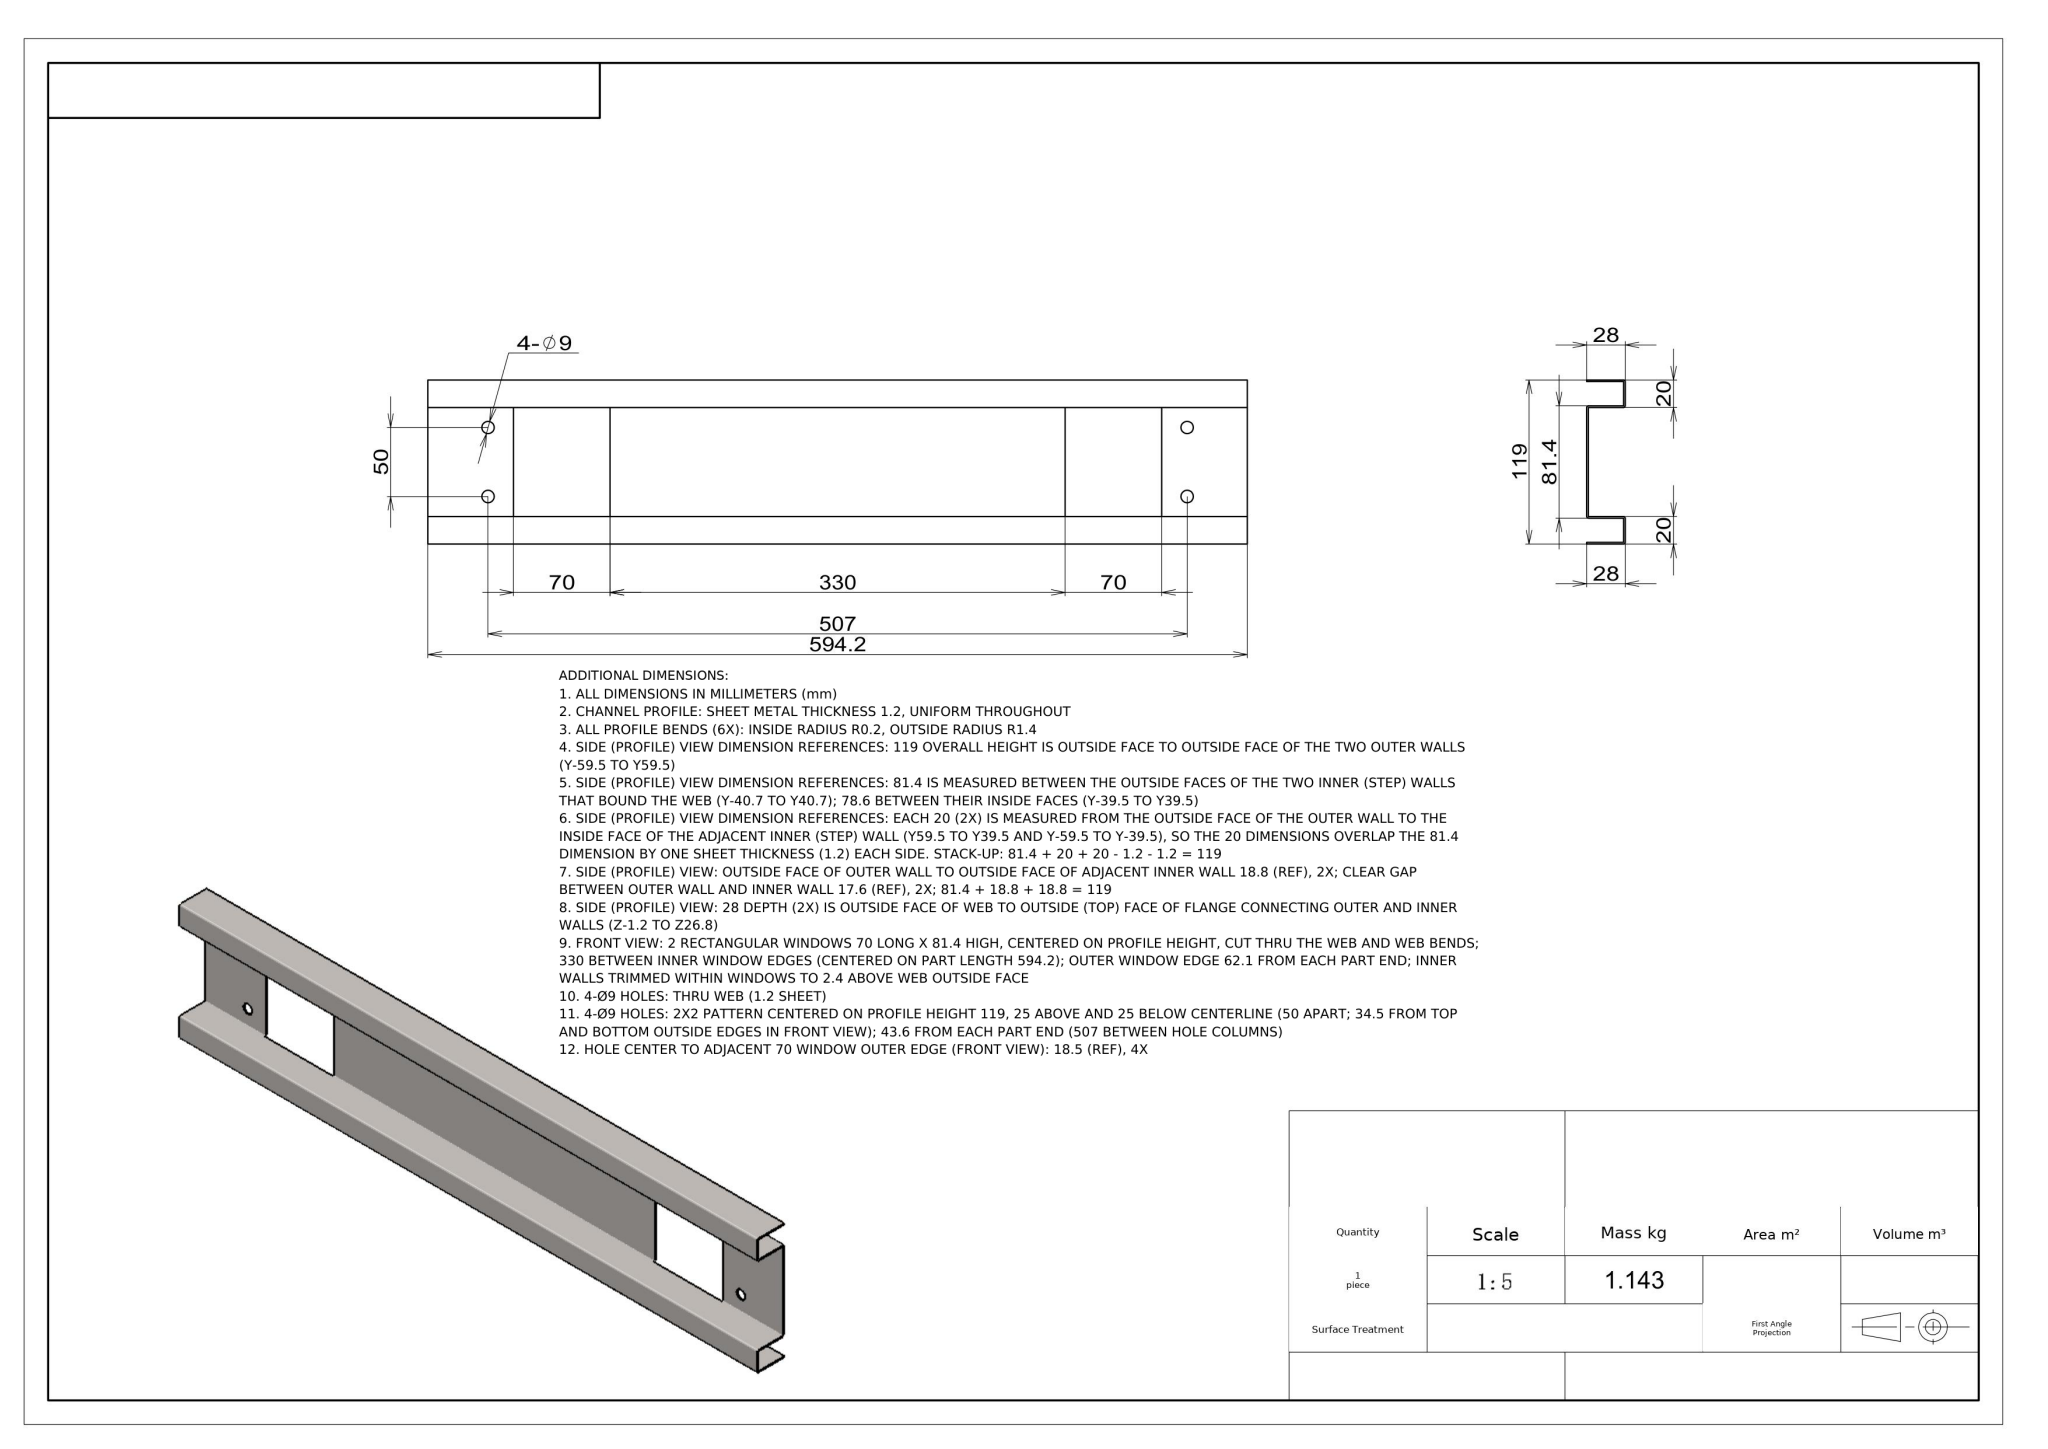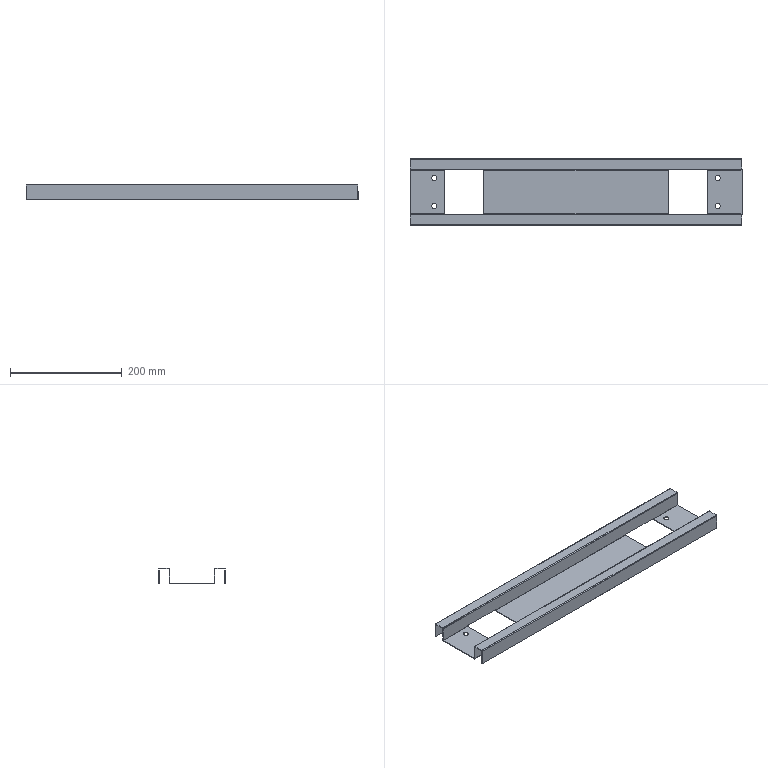Part | NX | mm | 1 solid | 98 faces | box 594.2 x 119 x 28 mm | volume 145552 mm3 | plane 70 | cylinder 28 | commonest cylinder face diameters 2.8 x10 0.4 x10 9 x8